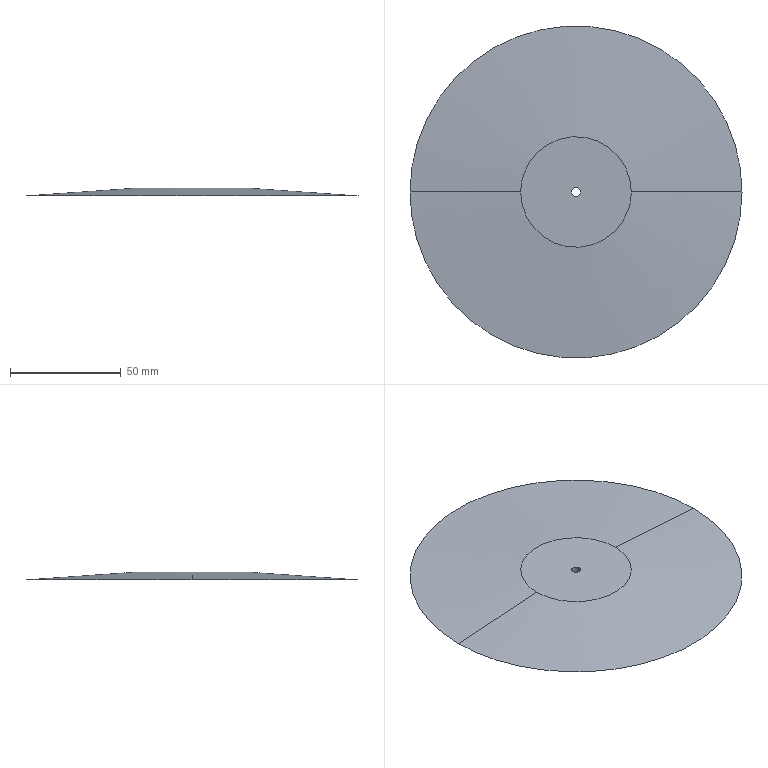CAM job | Mastercam | mm | 3 operations | part box 150 x 150 x 3.5
1. Surface Finish Flowline | 1 - 17 圆鼻铣刀
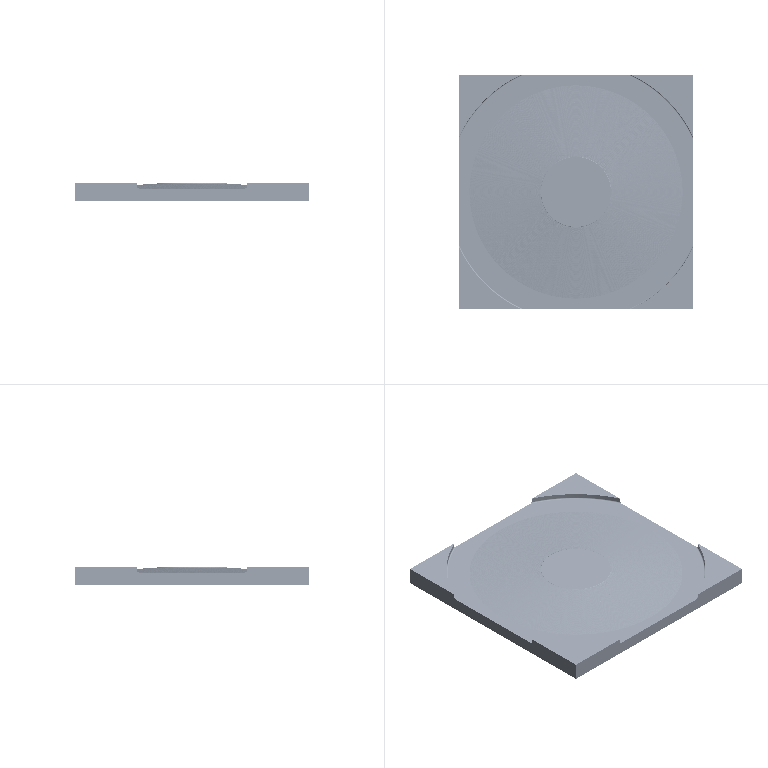2. Contour (Ramp) | 15 - 3 平铣刀
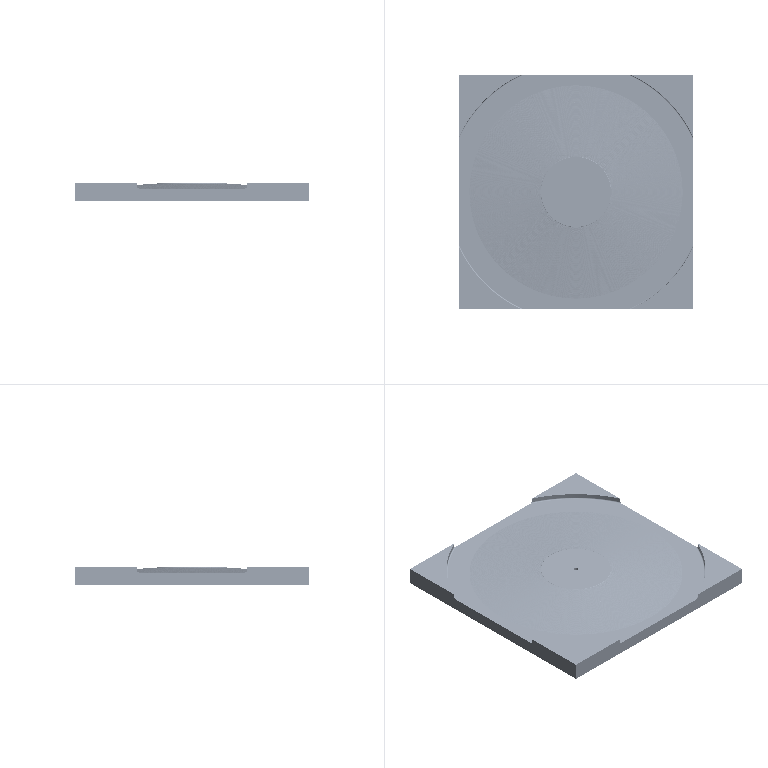3. Contour (2D) | 16 - 3 平铣刀